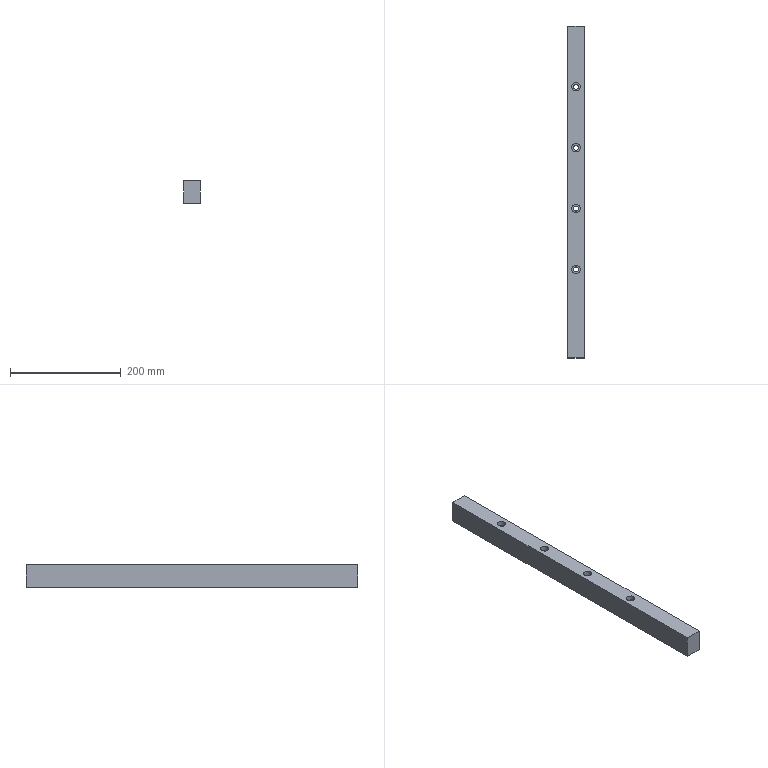Component | SolidWorks | GuideRailSpacer122-1 | 1 solid | 26 faces | box 30 x 600 x 41 mm | volume 723676 mm3 | cylinder 16 | plane 10 | commonest cylinder face diameters 15 x8 9 x8
build123d program:
from build123d import *

# Parameters (mm, degrees)
SKETCH1_W                                       = 30
SKETCH1_H                                       = 600
BOSS_EXTRUDE1_DEPTH                             = 41
M8_HEX_SOCKET_HEAD_CAP_SCREW_CBORE1_D           = 9
M8_HEX_SOCKET_HEAD_CAP_SCREW_CBORE1_CBORE_D     = 15
M8_HEX_SOCKET_HEAD_CAP_SCREW_CBORE1_CBORE_DEPTH = 8.6


with BuildPart() as part:
    # Sketch1 → Boss-Extrude1 (new body)
    with BuildSketch(Plane.XY):
        Rectangle(SKETCH1_W, SKETCH1_H)
    extrude(amount=BOSS_EXTRUDE1_DEPTH)

    # M8 Hex Socket Head Cap Screw CBORE1 (through all)
    with Locations(Plane.XY.offset(41)):
        with Locations((0, 190), (0, 80), (0, -30), (0, -140)):
            CounterBoreHole(M8_HEX_SOCKET_HEAD_CAP_SCREW_CBORE1_D / 2, M8_HEX_SOCKET_HEAD_CAP_SCREW_CBORE1_CBORE_D / 2, M8_HEX_SOCKET_HEAD_CAP_SCREW_CBORE1_CBORE_DEPTH)


solid = part.part

# Placed as in the assembly
solid = solid.moved(Location((-294.479, 164.741, 805), (0, 0, 0)))
STEP:
#1=COLOUR_RGB('',0.7922,0.8196,0.9333);
#2=FILL_AREA_STYLE_COLOUR('',#1);
#3=FILL_AREA_STYLE('',(#2));
#4=SURFACE_STYLE_FILL_AREA(#3);
#5=SURFACE_SIDE_STYLE('',(#4));
#6=SURFACE_STYLE_USAGE(.BOTH.,#5);
#7=PRESENTATION_STYLE_ASSIGNMENT((#6));
#8=CARTESIAN_POINT('',(-11.889,13.966,32.969));
#9=VERTEX_POINT('',#8);
#10=CARTESIAN_POINT('',(-11.298,13.966,32.969));
#11=VERTEX_POINT('',#10);
#12=CARTESIAN_POINT('',(-11.594,13.966,32.969));
#13=DIRECTION('',(0.,0.,1.));
#14=DIRECTION('',(1.,0.,0.));
#15=AXIS2_PLACEMENT_3D('',#12,#13,#14);
#16=CIRCLE('',#15,0.2953);
#17=EDGE_CURVE('',#9,#11,#16,.T.);
#18=ORIENTED_EDGE('',*,*,#17,.F.);
#19=CARTESIAN_POINT('',(-11.889,13.966,33.307));
#20=VERTEX_POINT('',#19);
#21=CARTESIAN_POINT('',(-11.889,13.966,33.307));
#22=DIRECTION('',(0.,0.,1.));
#23=VECTOR('',#22,39.37);
#24=LINE('',#21,#23);
#25=EDGE_CURVE('',#9,#20,#24,.T.);
#26=ORIENTED_EDGE('',*,*,#25,.T.);
#27=CARTESIAN_POINT('',(-11.298,13.966,33.307));
#28=VERTEX_POINT('',#27);
#29=CARTESIAN_POINT('',(-11.594,13.966,33.307));
#30=DIRECTION('',(0.,0.,1.));
#31=DIRECTION('',(1.,0.,0.));
#32=AXIS2_PLACEMENT_3D('',#29,#30,#31);
#33=CIRCLE('',#32,0.2953);
#34=EDGE_CURVE('',#20,#28,#33,.T.);
#35=ORIENTED_EDGE('',*,*,#34,.T.);
#36=CARTESIAN_POINT('',(-11.298,13.966,33.307));
#37=DIRECTION('',(0.,0.,1.));
#38=VECTOR('',#37,39.37);
#39=LINE('',#36,#38);
#40=EDGE_CURVE('',#11,#28,#39,.T.);
#41=ORIENTED_EDGE('',*,*,#40,.F.);
#42=EDGE_LOOP('',(#18,#26,#35,#41));
#43=FACE_OUTER_BOUND('',#42,.T.);
#44=CARTESIAN_POINT('',(-11.594,13.966,33.307));
#45=DIRECTION('',(0.,0.,1.));
#46=DIRECTION('',(1.,0.,0.));
#47=AXIS2_PLACEMENT_3D('',#44,#45,#46);
#48=CYLINDRICAL_SURFACE('',#47,0.2953);
#49=ADVANCED_FACE('',(#43),#48,.F.);
#50=CARTESIAN_POINT('',(-11.771,13.966,31.693));
#51=VERTEX_POINT('',#50);
#52=CARTESIAN_POINT('',(-11.416,13.966,31.693));
#53=VERTEX_POINT('',#52);
#54=CARTESIAN_POINT('',(-11.594,13.966,31.693));
#55=DIRECTION('',(0.,0.,1.));
#56=DIRECTION('',(1.,0.,0.));
#57=AXIS2_PLACEMENT_3D('',#54,#55,#56);
#58=CIRCLE('',#57,0.1772);
#59=EDGE_CURVE('',#51,#53,#58,.T.);
#60=ORIENTED_EDGE('',*,*,#59,.F.);
#61=CARTESIAN_POINT('',(-11.771,13.966,32.969));
#62=VERTEX_POINT('',#61);
#63=CARTESIAN_POINT('',(-11.771,13.966,33.307));
#64=DIRECTION('',(0.,0.,1.));
#65=VECTOR('',#64,39.37);
#66=LINE('',#63,#65);
#67=EDGE_CURVE('',#51,#62,#66,.T.);
#68=ORIENTED_EDGE('',*,*,#67,.T.);
#69=CARTESIAN_POINT('',(-11.416,13.966,32.969));
#70=VERTEX_POINT('',#69);
#71=CARTESIAN_POINT('',(-11.594,13.966,32.969));
#72=DIRECTION('',(0.,0.,1.));
#73=DIRECTION('',(1.,0.,0.));
#74=AXIS2_PLACEMENT_3D('',#71,#72,#73);
#75=CIRCLE('',#74,0.1772);
#76=EDGE_CURVE('',#62,#70,#75,.T.);
#77=ORIENTED_EDGE('',*,*,#76,.T.);
#78=CARTESIAN_POINT('',(-11.416,13.966,33.307));
#79=DIRECTION('',(0.,0.,1.));
#80=VECTOR('',#79,39.37);
#81=LINE('',#78,#80);
#82=EDGE_CURVE('',#53,#70,#81,.T.);
#83=ORIENTED_EDGE('',*,*,#82,.F.);
#84=EDGE_LOOP('',(#60,#68,#77,#83));
#85=FACE_OUTER_BOUND('',#84,.T.);
#86=CARTESIAN_POINT('',(-11.594,13.966,33.307));
#87=DIRECTION('',(0.,0.,1.));
#88=DIRECTION('',(1.,0.,0.));
#89=AXIS2_PLACEMENT_3D('',#86,#87,#88);
#90=CYLINDRICAL_SURFACE('',#89,0.1772);
#91=ADVANCED_FACE('',(#85),#90,.F.);
#92=CARTESIAN_POINT('',(-11.889,9.635,32.969));
#93=VERTEX_POINT('',#92);
#94=CARTESIAN_POINT('',(-11.298,9.635,32.969));
#95=VERTEX_POINT('',#94);
#96=CARTESIAN_POINT('',(-11.594,9.635,32.969));
#97=DIRECTION('',(0.,0.,1.));
#98=DIRECTION('',(1.,0.,0.));
#99=AXIS2_PLACEMENT_3D('',#96,#97,#98);
#100=CIRCLE('',#99,0.2953);
#101=EDGE_CURVE('',#93,#95,#100,.T.);
#102=ORIENTED_EDGE('',*,*,#101,.F.);
#103=CARTESIAN_POINT('',(-11.889,9.635,33.307));
#104=VERTEX_POINT('',#103);
#105=CARTESIAN_POINT('',(-11.889,9.635,33.307));
#106=DIRECTION('',(0.,0.,1.));
#107=VECTOR('',#106,39.37);
#108=LINE('',#105,#107);
#109=EDGE_CURVE('',#93,#104,#108,.T.);
#110=ORIENTED_EDGE('',*,*,#109,.T.);
#111=CARTESIAN_POINT('',(-11.298,9.635,33.307));
#112=VERTEX_POINT('',#111);
#113=CARTESIAN_POINT('',(-11.594,9.635,33.307));
#114=DIRECTION('',(0.,0.,1.));
#115=DIRECTION('',(1.,0.,0.));
#116=AXIS2_PLACEMENT_3D('',#113,#114,#115);
#117=CIRCLE('',#116,0.2953);
#118=EDGE_CURVE('',#104,#112,#117,.T.);
#119=ORIENTED_EDGE('',*,*,#118,.T.);
#120=CARTESIAN_POINT('',(-11.298,9.635,33.307));
#121=DIRECTION('',(0.,0.,1.));
#122=VECTOR('',#121,39.37);
#123=LINE('',#120,#122);
#124=EDGE_CURVE('',#95,#112,#123,.T.);
#125=ORIENTED_EDGE('',*,*,#124,.F.);
#126=EDGE_LOOP('',(#102,#110,#119,#125));
#127=FACE_OUTER_BOUND('',#126,.T.);
#128=CARTESIAN_POINT('',(-11.594,9.635,33.307));
#129=DIRECTION('',(0.,0.,1.));
#130=DIRECTION('',(1.,0.,0.));
#131=AXIS2_PLACEMENT_3D('',#128,#129,#130);
#132=CYLINDRICAL_SURFACE('',#131,0.2953);
#133=ADVANCED_FACE('',(#127),#132,.F.);
#134=CARTESIAN_POINT('',(-11.771,9.635,31.693));
#135=VERTEX_POINT('',#134);
#136=CARTESIAN_POINT('',(-11.416,9.635,31.693));
#137=VERTEX_POINT('',#136);
#138=CARTESIAN_POINT('',(-11.594,9.635,31.693));
#139=DIRECTION('',(0.,0.,1.));
#140=DIRECTION('',(1.,0.,0.));
#141=AXIS2_PLACEMENT_3D('',#138,#139,#140);
#142=CIRCLE('',#141,0.1772);
#143=EDGE_CURVE('',#135,#137,#142,.T.);
#144=ORIENTED_EDGE('',*,*,#143,.F.);
#145=CARTESIAN_POINT('',(-11.771,9.635,32.969));
#146=VERTEX_POINT('',#145);
#147=CARTESIAN_POINT('',(-11.771,9.635,33.307));
#148=DIRECTION('',(0.,0.,1.));
#149=VECTOR('',#148,39.37);
#150=LINE('',#147,#149);
#151=EDGE_CURVE('',#135,#146,#150,.T.);
#152=ORIENTED_EDGE('',*,*,#151,.T.);
#153=CARTESIAN_POINT('',(-11.416,9.635,32.969));
#154=VERTEX_POINT('',#153);
#155=CARTESIAN_POINT('',(-11.594,9.635,32.969));
#156=DIRECTION('',(0.,0.,1.));
#157=DIRECTION('',(1.,0.,0.));
#158=AXIS2_PLACEMENT_3D('',#155,#156,#157);
#159=CIRCLE('',#158,0.1772);
#160=EDGE_CURVE('',#146,#154,#159,.T.);
#161=ORIENTED_EDGE('',*,*,#160,.T.);
#162=CARTESIAN_POINT('',(-11.416,9.635,33.307));
#163=DIRECTION('',(0.,0.,1.));
#164=VECTOR('',#163,39.37);
#165=LINE('',#162,#164);
#166=EDGE_CURVE('',#137,#154,#165,.T.);
#167=ORIENTED_EDGE('',*,*,#166,.F.);
#168=EDGE_LOOP('',(#144,#152,#161,#167));
#169=FACE_OUTER_BOUND('',#168,.T.);
#170=CARTESIAN_POINT('',(-11.594,9.635,33.307));
#171=DIRECTION('',(0.,0.,1.));
#172=DIRECTION('',(1.,0.,0.));
#173=AXIS2_PLACEMENT_3D('',#170,#171,#172);
#174=CYLINDRICAL_SURFACE('',#173,0.1772);
#175=ADVANCED_FACE('',(#169),#174,.F.);
#176=CARTESIAN_POINT('',(-11.889,5.305,32.969));
#177=VERTEX_POINT('',#176);
#178=CARTESIAN_POINT('',(-11.298,5.305,32.969));
#179=VERTEX_POINT('',#178);
#180=CARTESIAN_POINT('',(-11.594,5.305,32.969));
#181=DIRECTION('',(0.,0.,1.));
#182=DIRECTION('',(1.,0.,0.));
#183=AXIS2_PLACEMENT_3D('',#180,#181,#182);
#184=CIRCLE('',#183,0.2953);
#185=EDGE_CURVE('',#177,#179,#184,.T.);
#186=ORIENTED_EDGE('',*,*,#185,.F.);
#187=CARTESIAN_POINT('',(-11.889,5.305,33.307));
#188=VERTEX_POINT('',#187);
#189=CARTESIAN_POINT('',(-11.889,5.305,33.307));
#190=DIRECTION('',(0.,0.,1.));
#191=VECTOR('',#190,39.37);
#192=LINE('',#189,#191);
#193=EDGE_CURVE('',#177,#188,#192,.T.);
#194=ORIENTED_EDGE('',*,*,#193,.T.);
#195=CARTESIAN_POINT('',(-11.298,5.305,33.307));
#196=VERTEX_POINT('',#195);
#197=CARTESIAN_POINT('',(-11.594,5.305,33.307));
#198=DIRECTION('',(0.,0.,1.));
#199=DIRECTION('',(1.,0.,0.));
#200=AXIS2_PLACEMENT_3D('',#197,#198,#199);
#201=CIRCLE('',#200,0.2953);
#202=EDGE_CURVE('',#188,#196,#201,.T.);
#203=ORIENTED_EDGE('',*,*,#202,.T.);
#204=CARTESIAN_POINT('',(-11.298,5.305,33.307));
#205=DIRECTION('',(0.,0.,1.));
#206=VECTOR('',#205,39.37);
#207=LINE('',#204,#206);
#208=EDGE_CURVE('',#179,#196,#207,.T.);
#209=ORIENTED_EDGE('',*,*,#208,.F.);
#210=EDGE_LOOP('',(#186,#194,#203,#209));
#211=FACE_OUTER_BOUND('',#210,.T.);
#212=CARTESIAN_POINT('',(-11.594,5.305,33.307));
#213=DIRECTION('',(0.,0.,1.));
#214=DIRECTION('',(1.,0.,0.));
#215=AXIS2_PLACEMENT_3D('',#212,#213,#214);
#216=CYLINDRICAL_SURFACE('',#215,0.2953);
#217=ADVANCED_FACE('',(#211),#216,.F.);
#218=CARTESIAN_POINT('',(-11.771,5.305,31.693));
#219=VERTEX_POINT('',#218);
#220=CARTESIAN_POINT('',(-11.416,5.305,31.693));
#221=VERTEX_POINT('',#220);
#222=CARTESIAN_POINT('',(-11.594,5.305,31.693));
#223=DIRECTION('',(0.,0.,1.));
#224=DIRECTION('',(1.,0.,0.));
#225=AXIS2_PLACEMENT_3D('',#222,#223,#224);
#226=CIRCLE('',#225,0.1772);
#227=EDGE_CURVE('',#219,#221,#226,.T.);
#228=ORIENTED_EDGE('',*,*,#227,.F.);
#229=CARTESIAN_POINT('',(-11.771,5.305,32.969));
#230=VERTEX_POINT('',#229);
#231=CARTESIAN_POINT('',(-11.771,5.305,33.307));
#232=DIRECTION('',(0.,0.,1.));
#233=VECTOR('',#232,39.37);
#234=LINE('',#231,#233);
#235=EDGE_CURVE('',#219,#230,#234,.T.);
#236=ORIENTED_EDGE('',*,*,#235,.T.);
#237=CARTESIAN_POINT('',(-11.416,5.305,32.969));
#238=VERTEX_POINT('',#237);
#239=CARTESIAN_POINT('',(-11.594,5.305,32.969));
#240=DIRECTION('',(0.,0.,1.));
#241=DIRECTION('',(1.,0.,0.));
#242=AXIS2_PLACEMENT_3D('',#239,#240,#241);
#243=CIRCLE('',#242,0.1772);
#244=EDGE_CURVE('',#230,#238,#243,.T.);
#245=ORIENTED_EDGE('',*,*,#244,.T.);
#246=CARTESIAN_POINT('',(-11.416,5.305,33.307));
#247=DIRECTION('',(0.,0.,1.));
#248=VECTOR('',#247,39.37);
#249=LINE('',#246,#248);
#250=EDGE_CURVE('',#221,#238,#249,.T.);
#251=ORIENTED_EDGE('',*,*,#250,.F.);
#252=EDGE_LOOP('',(#228,#236,#245,#251));
#253=FACE_OUTER_BOUND('',#252,.T.);
#254=CARTESIAN_POINT('',(-11.594,5.305,33.307));
#255=DIRECTION('',(0.,0.,1.));
#256=DIRECTION('',(1.,0.,0.));
#257=AXIS2_PLACEMENT_3D('',#254,#255,#256);
#258=CYLINDRICAL_SURFACE('',#257,0.1772);
#259=ADVANCED_FACE('',(#253),#258,.F.);
#260=CARTESIAN_POINT('',(-11.889,0.974,32.969));
#261=VERTEX_POINT('',#260);
#262=CARTESIAN_POINT('',(-11.298,0.974,32.969));
#263=VERTEX_POINT('',#262);
#264=CARTESIAN_POINT('',(-11.594,0.974,32.969));
#265=DIRECTION('',(0.,0.,1.));
#266=DIRECTION('',(1.,0.,0.));
#267=AXIS2_PLACEMENT_3D('',#264,#265,#266);
#268=CIRCLE('',#267,0.2953);
#269=EDGE_CURVE('',#261,#263,#268,.T.);
#270=ORIENTED_EDGE('',*,*,#269,.F.);
#271=CARTESIAN_POINT('',(-11.889,0.974,33.307));
#272=VERTEX_POINT('',#271);
#273=CARTESIAN_POINT('',(-11.889,0.974,33.307));
#274=DIRECTION('',(0.,0.,1.));
#275=VECTOR('',#274,39.37);
#276=LINE('',#273,#275);
#277=EDGE_CURVE('',#261,#272,#276,.T.);
#278=ORIENTED_EDGE('',*,*,#277,.T.);
#279=CARTESIAN_POINT('',(-11.298,0.974,33.307));
#280=VERTEX_POINT('',#279);
#281=CARTESIAN_POINT('',(-11.594,0.974,33.307));
#282=DIRECTION('',(0.,0.,1.));
#283=DIRECTION('',(1.,0.,0.));
#284=AXIS2_PLACEMENT_3D('',#281,#282,#283);
#285=CIRCLE('',#284,0.2953);
#286=EDGE_CURVE('',#272,#280,#285,.T.);
#287=ORIENTED_EDGE('',*,*,#286,.T.);
#288=CARTESIAN_POINT('',(-11.298,0.974,33.307));
#289=DIRECTION('',(0.,0.,1.));
#290=VECTOR('',#289,39.37);
#291=LINE('',#288,#290);
#292=EDGE_CURVE('',#263,#280,#291,.T.);
#293=ORIENTED_EDGE('',*,*,#292,.F.);
#294=EDGE_LOOP('',(#270,#278,#287,#293));
#295=FACE_OUTER_BOUND('',#294,.T.);
#296=CARTESIAN_POINT('',(-11.594,0.974,33.307));
#297=DIRECTION('',(0.,0.,1.));
#298=DIRECTION('',(1.,0.,0.));
#299=AXIS2_PLACEMENT_3D('',#296,#297,#298);
#300=CYLINDRICAL_SURFACE('',#299,0.2953);
#301=ADVANCED_FACE('',(#295),#300,.F.);
#302=CARTESIAN_POINT('',(-11.771,0.974,31.693));
#303=VERTEX_POINT('',#302);
#304=CARTESIAN_POINT('',(-11.416,0.974,31.693));
#305=VERTEX_POINT('',#304);
#306=CARTESIAN_POINT('',(-11.594,0.974,31.693));
#307=DIRECTION('',(0.,0.,1.));
#308=DIRECTION('',(1.,0.,0.));
#309=AXIS2_PLACEMENT_3D('',#306,#307,#308);
#310=CIRCLE('',#309,0.1772);
#311=EDGE_CURVE('',#303,#305,#310,.T.);
#312=ORIENTED_EDGE('',*,*,#311,.F.);
#313=CARTESIAN_POINT('',(-11.771,0.974,32.969));
#314=VERTEX_POINT('',#313);
#315=CARTESIAN_POINT('',(-11.771,0.974,33.307));
#316=DIRECTION('',(0.,0.,1.));
#317=VECTOR('',#316,39.37);
#318=LINE('',#315,#317);
#319=EDGE_CURVE('',#303,#314,#318,.T.);
#320=ORIENTED_EDGE('',*,*,#319,.T.);
#321=CARTESIAN_POINT('',(-11.416,0.974,32.969));
#322=VERTEX_POINT('',#321);
#323=CARTESIAN_POINT('',(-11.594,0.974,32.969));
#324=DIRECTION('',(0.,0.,1.));
#325=DIRECTION('',(1.,0.,0.));
#326=AXIS2_PLACEMENT_3D('',#323,#324,#325);
#327=CIRCLE('',#326,0.1772);
#328=EDGE_CURVE('',#314,#322,#327,.T.);
#329=ORIENTED_EDGE('',*,*,#328,.T.);
#330=CARTESIAN_POINT('',(-11.416,0.974,33.307));
#331=DIRECTION('',(0.,0.,1.));
#332=VECTOR('',#331,39.37);
#333=LINE('',#330,#332);
#334=EDGE_CURVE('',#305,#322,#333,.T.);
#335=ORIENTED_EDGE('',*,*,#334,.F.);
#336=EDGE_LOOP('',(#312,#320,#329,#335));
#337=FACE_OUTER_BOUND('',#336,.T.);
#338=CARTESIAN_POINT('',(-11.594,0.974,33.307));
#339=DIRECTION('',(0.,0.,1.));
#340=DIRECTION('',(1.,0.,0.));
#341=AXIS2_PLACEMENT_3D('',#338,#339,#340);
#342=CYLINDRICAL_SURFACE('',#341,0.1772);
#343=ADVANCED_FACE('',(#337),#342,.F.);
#344=CARTESIAN_POINT('',(-11.003,-5.325,31.693));
#345=VERTEX_POINT('',#344);
#346=CARTESIAN_POINT('',(-11.003,18.297,31.693));
#347=VERTEX_POINT('',#346);
#348=CARTESIAN_POINT('',(-11.003,-5.325,31.693));
#349=DIRECTION('',(0.,1.,0.));
#350=VECTOR('',#349,39.37);
#351=LINE('',#348,#350);
#352=EDGE_CURVE('',#345,#347,#351,.T.);
#353=ORIENTED_EDGE('',*,*,#352,.T.);
#354=CARTESIAN_POINT('',(-11.003,18.297,33.307));
#355=VERTEX_POINT('',#354);
#356=CARTESIAN_POINT('',(-11.003,18.297,33.307));
#357=DIRECTION('',(0.,0.,-1.));
#358=VECTOR('',#357,39.37);
#359=LINE('',#356,#358);
#360=EDGE_CURVE('',#355,#347,#359,.T.);
#361=ORIENTED_EDGE('',*,*,#360,.F.);
#362=CARTESIAN_POINT('',(-11.003,-5.325,33.307));
#363=VERTEX_POINT('',#362);
#364=CARTESIAN_POINT('',(-11.003,-5.325,33.307));
#365=DIRECTION('',(0.,1.,0.));
#366=VECTOR('',#365,39.37);
#367=LINE('',#364,#366);
#368=EDGE_CURVE('',#363,#355,#367,.T.);
#369=ORIENTED_EDGE('',*,*,#368,.F.);
#370=CARTESIAN_POINT('',(-11.003,-5.325,33.307));
#371=DIRECTION('',(0.,0.,-1.));
#372=VECTOR('',#371,39.37);
#373=LINE('',#370,#372);
#374=EDGE_CURVE('',#363,#345,#373,.T.);
#375=ORIENTED_EDGE('',*,*,#374,.T.);
#376=EDGE_LOOP('',(#353,#361,#369,#375));
#377=FACE_OUTER_BOUND('',#376,.T.);
#378=CARTESIAN_POINT('',(-11.003,-5.325,33.307));
#379=DIRECTION('',(-1.,0.,0.));
#380=DIRECTION('',(0.,0.,1.));
#381=AXIS2_PLACEMENT_3D('',#378,#379,#380);
#382=PLANE('',#381);
#383=ADVANCED_FACE('',(#377),#382,.F.);
#384=CARTESIAN_POINT('',(-12.184,18.297,31.693));
#385=VERTEX_POINT('',#384);
#386=CARTESIAN_POINT('',(-12.184,18.297,31.693));
#387=DIRECTION('',(-1.,0.,0.));
#388=VECTOR('',#387,39.37);
#389=LINE('',#386,#388);
#390=EDGE_CURVE('',#347,#385,#389,.T.);
#391=ORIENTED_EDGE('',*,*,#390,.T.);
#392=CARTESIAN_POINT('',(-12.184,18.297,33.307));
#393=VERTEX_POINT('',#392);
#394=CARTESIAN_POINT('',(-12.184,18.297,33.307));
#395=DIRECTION('',(0.,0.,-1.));
#396=VECTOR('',#395,39.37);
#397=LINE('',#394,#396);
#398=EDGE_CURVE('',#393,#385,#397,.T.);
#399=ORIENTED_EDGE('',*,*,#398,.F.);
#400=CARTESIAN_POINT('',(-12.184,18.297,33.307));
#401=DIRECTION('',(-1.,0.,0.));
#402=VECTOR('',#401,39.37);
#403=LINE('',#400,#402);
#404=EDGE_CURVE('',#355,#393,#403,.T.);
#405=ORIENTED_EDGE('',*,*,#404,.F.);
#406=ORIENTED_EDGE('',*,*,#360,.T.);
#407=EDGE_LOOP('',(#391,#399,#405,#406));
#408=FACE_OUTER_BOUND('',#407,.T.);
#409=CARTESIAN_POINT('',(-12.184,18.297,33.307));
#410=DIRECTION('',(0.,-1.,0.));
#411=DIRECTION('',(0.,0.,-1.));
#412=AXIS2_PLACEMENT_3D('',#409,#410,#411);
#413=PLANE('',#412);
#414=ADVANCED_FACE('',(#408),#413,.F.);
#415=CARTESIAN_POINT('',(-12.184,-5.325,31.693));
#416=VERTEX_POINT('',#415);
#417=CARTESIAN_POINT('',(-12.184,-5.325,31.693));
#418=DIRECTION('',(0.,-1.,0.));
#419=VECTOR('',#418,39.37);
#420=LINE('',#417,#419);
#421=EDGE_CURVE('',#385,#416,#420,.T.);
#422=ORIENTED_EDGE('',*,*,#421,.T.);
#423=CARTESIAN_POINT('',(-12.184,-5.325,33.307));
#424=VERTEX_POINT('',#423);
#425=CARTESIAN_POINT('',(-12.184,-5.325,33.307));
#426=DIRECTION('',(0.,0.,-1.));
#427=VECTOR('',#426,39.37);
#428=LINE('',#425,#427);
#429=EDGE_CURVE('',#424,#416,#428,.T.);
#430=ORIENTED_EDGE('',*,*,#429,.F.);
#431=CARTESIAN_POINT('',(-12.184,-5.325,33.307));
#432=DIRECTION('',(0.,-1.,0.));
#433=VECTOR('',#432,39.37);
#434=LINE('',#431,#433);
#435=EDGE_CURVE('',#393,#424,#434,.T.);
#436=ORIENTED_EDGE('',*,*,#435,.F.);
#437=ORIENTED_EDGE('',*,*,#398,.T.);
#438=EDGE_LOOP('',(#422,#430,#436,#437));
#439=FACE_OUTER_BOUND('',#438,.T.);
#440=CARTESIAN_POINT('',(-12.184,-5.325,33.307));
#441=DIRECTION('',(1.,0.,0.));
#442=DIRECTION('',(0.,0.,-1.));
#443=AXIS2_PLACEMENT_3D('',#440,#441,#442);
#444=PLANE('',#443);
#445=ADVANCED_FACE('',(#439),#444,.F.);
#446=CARTESIAN_POINT('',(-12.184,-5.325,31.693));
#447=DIRECTION('',(1.,0.,0.));
#448=VECTOR('',#447,39.37);
#449=LINE('',#446,#448);
#450=EDGE_CURVE('',#416,#345,#449,.T.);
#451=ORIENTED_EDGE('',*,*,#450,.T.);
#452=ORIENTED_EDGE('',*,*,#374,.F.);
#453=CARTESIAN_POINT('',(-12.184,-5.325,33.307));
#454=DIRECTION('',(1.,0.,0.));
#455=VECTOR('',#454,39.37);
#456=LINE('',#453,#455);
#457=EDGE_CURVE('',#424,#363,#456,.T.);
#458=ORIENTED_EDGE('',*,*,#457,.F.);
#459=ORIENTED_EDGE('',*,*,#429,.T.);
#460=EDGE_LOOP('',(#451,#452,#458,#459));
#461=FACE_OUTER_BOUND('',#460,.T.);
#462=CARTESIAN_POINT('',(-12.184,-5.325,33.307));
#463=DIRECTION('',(0.,1.,0.));
#464=DIRECTION('',(0.,0.,1.));
#465=AXIS2_PLACEMENT_3D('',#462,#463,#464);
#466=PLANE('',#465);
#467=ADVANCED_FACE('',(#461),#466,.F.);
#468=CARTESIAN_POINT('',(-11.594,13.966,33.307));
#469=DIRECTION('',(0.,0.,1.));
#470=DIRECTION('',(1.,0.,0.));
#471=AXIS2_PLACEMENT_3D('',#468,#469,#470);
#472=CIRCLE('',#471,0.2953);
#473=EDGE_CURVE('',#28,#20,#472,.T.);
#474=ORIENTED_EDGE('',*,*,#473,.F.);
#475=ORIENTED_EDGE('',*,*,#34,.F.);
#476=EDGE_LOOP('',(#474,#475));
#477=FACE_BOUND('',#476,.T.);
#478=CARTESIAN_POINT('',(-11.594,9.635,33.307));
#479=DIRECTION('',(0.,0.,1.));
#480=DIRECTION('',(1.,0.,0.));
#481=AXIS2_PLACEMENT_3D('',#478,#479,#480);
#482=CIRCLE('',#481,0.2953);
#483=EDGE_CURVE('',#112,#104,#482,.T.);
#484=ORIENTED_EDGE('',*,*,#483,.F.);
#485=ORIENTED_EDGE('',*,*,#118,.F.);
#486=EDGE_LOOP('',(#484,#485));
#487=FACE_BOUND('',#486,.T.);
#488=CARTESIAN_POINT('',(-11.594,5.305,33.307));
#489=DIRECTION('',(0.,0.,1.));
#490=DIRECTION('',(1.,0.,0.));
#491=AXIS2_PLACEMENT_3D('',#488,#489,#490);
#492=CIRCLE('',#491,0.2953);
#493=EDGE_CURVE('',#196,#188,#492,.T.);
#494=ORIENTED_EDGE('',*,*,#493,.F.);
#495=ORIENTED_EDGE('',*,*,#202,.F.);
#496=EDGE_LOOP('',(#494,#495));
#497=FACE_BOUND('',#496,.T.);
#498=CARTESIAN_POINT('',(-11.594,0.974,33.307));
#499=DIRECTION('',(0.,0.,1.));
#500=DIRECTION('',(1.,0.,0.));
#501=AXIS2_PLACEMENT_3D('',#498,#499,#500);
#502=CIRCLE('',#501,0.2953);
#503=EDGE_CURVE('',#280,#272,#502,.T.);
#504=ORIENTED_EDGE('',*,*,#503,.F.);
#505=ORIENTED_EDGE('',*,*,#286,.F.);
#506=EDGE_LOOP('',(#504,#505));
#507=FACE_BOUND('',#506,.T.);
#508=ORIENTED_EDGE('',*,*,#368,.T.);
#509=ORIENTED_EDGE('',*,*,#404,.T.);
#510=ORIENTED_EDGE('',*,*,#435,.T.);
#511=ORIENTED_EDGE('',*,*,#457,.T.);
#512=EDGE_LOOP('',(#508,#509,#510,#511));
#513=FACE_OUTER_BOUND('',#512,.T.);
#514=CARTESIAN_POINT('',(-11.594,6.486,33.307));
#515=DIRECTION('',(0.,0.,-1.));
#516=DIRECTION('',(-1.,0.,0.));
#517=AXIS2_PLACEMENT_3D('',#514,#515,#516);
#518=PLANE('',#517);
#519=ADVANCED_FACE('',(#477,#487,#497,#507,#513),#518,.F.);
#520=CARTESIAN_POINT('',(-11.594,13.966,31.693));
#521=DIRECTION('',(0.,0.,1.));
#522=DIRECTION('',(1.,0.,0.));
#523=AXIS2_PLACEMENT_3D('',#520,#521,#522);
#524=CIRCLE('',#523,0.1772);
#525=EDGE_CURVE('',#53,#51,#524,.T.);
#526=ORIENTED_EDGE('',*,*,#525,.T.);
#527=ORIENTED_EDGE('',*,*,#59,.T.);
#528=EDGE_LOOP('',(#526,#527));
#529=FACE_BOUND('',#528,.T.);
#530=CARTESIAN_POINT('',(-11.594,9.635,31.693));
#531=DIRECTION('',(0.,0.,1.));
#532=DIRECTION('',(1.,0.,0.));
#533=AXIS2_PLACEMENT_3D('',#530,#531,#532);
#534=CIRCLE('',#533,0.1772);
#535=EDGE_CURVE('',#137,#135,#534,.T.);
#536=ORIENTED_EDGE('',*,*,#535,.T.);
#537=ORIENTED_EDGE('',*,*,#143,.T.);
#538=EDGE_LOOP('',(#536,#537));
#539=FACE_BOUND('',#538,.T.);
#540=CARTESIAN_POINT('',(-11.594,5.305,31.693));
#541=DIRECTION('',(0.,0.,1.));
#542=DIRECTION('',(1.,0.,0.));
#543=AXIS2_PLACEMENT_3D('',#540,#541,#542);
#544=CIRCLE('',#543,0.1772);
#545=EDGE_CURVE('',#221,#219,#544,.T.);
#546=ORIENTED_EDGE('',*,*,#545,.T.);
#547=ORIENTED_EDGE('',*,*,#227,.T.);
#548=EDGE_LOOP('',(#546,#547));
#549=FACE_BOUND('',#548,.T.);
#550=CARTESIAN_POINT('',(-11.594,0.974,31.693));
#551=DIRECTION('',(0.,0.,1.));
#552=DIRECTION('',(1.,0.,0.));
#553=AXIS2_PLACEMENT_3D('',#550,#551,#552);
#554=CIRCLE('',#553,0.1772);
#555=EDGE_CURVE('',#305,#303,#554,.T.);
#556=ORIENTED_EDGE('',*,*,#555,.T.);
#557=ORIENTED_EDGE('',*,*,#311,.T.);
#558=EDGE_LOOP('',(#556,#557));
#559=FACE_BOUND('',#558,.T.);
#560=ORIENTED_EDGE('',*,*,#352,.F.);
#561=ORIENTED_EDGE('',*,*,#450,.F.);
#562=ORIENTED_EDGE('',*,*,#421,.F.);
#563=ORIENTED_EDGE('',*,*,#390,.F.);
#564=EDGE_LOOP('',(#560,#561,#562,#563));
#565=FACE_OUTER_BOUND('',#564,.T.);
#566=CARTESIAN_POINT('',(-11.594,6.486,31.693));
#567=DIRECTION('',(0.,0.,-1.));
#568=DIRECTION('',(-1.,0.,0.));
#569=AXIS2_PLACEMENT_3D('',#566,#567,#568);
#570=PLANE('',#569);
#571=ADVANCED_FACE('',(#529,#539,#549,#559,#565),#570,.T.);
#572=ORIENTED_EDGE('',*,*,#319,.F.);
#573=ORIENTED_EDGE('',*,*,#555,.F.);
#574=ORIENTED_EDGE('',*,*,#334,.T.);
#575=CARTESIAN_POINT('',(-11.594,0.974,32.969));
#576=DIRECTION('',(0.,0.,1.));
#577=DIRECTION('',(1.,0.,0.));
#578=AXIS2_PLACEMENT_3D('',#575,#576,#577);
#579=CIRCLE('',#578,0.1772);
#580=EDGE_CURVE('',#322,#314,#579,.T.);
#581=ORIENTED_EDGE('',*,*,#580,.T.);
#582=EDGE_LOOP('',(#572,#573,#574,#581));
#583=FACE_OUTER_BOUND('',#582,.T.);
#584=CARTESIAN_POINT('',(-11.594,0.974,33.307));
#585=DIRECTION('',(0.,0.,1.));
#586=DIRECTION('',(1.,0.,0.));
#587=AXIS2_PLACEMENT_3D('',#584,#585,#586);
#588=CYLINDRICAL_SURFACE('',#587,0.1772);
#589=ADVANCED_FACE('',(#583),#588,.F.);
#590=ORIENTED_EDGE('',*,*,#580,.F.);
#591=ORIENTED_EDGE('',*,*,#328,.F.);
#592=EDGE_LOOP('',(#590,#591));
#593=FACE_BOUND('',#592,.T.);
#594=CARTESIAN_POINT('',(-11.594,0.974,32.969));
#595=DIRECTION('',(0.,0.,1.));
#596=DIRECTION('',(1.,0.,0.));
#597=AXIS2_PLACEMENT_3D('',#594,#595,#596);
#598=CIRCLE('',#597,0.2953);
#599=EDGE_CURVE('',#263,#261,#598,.T.);
#600=ORIENTED_EDGE('',*,*,#599,.T.);
#601=ORIENTED_EDGE('',*,*,#269,.T.);
#602=EDGE_LOOP('',(#600,#601));
#603=FACE_OUTER_BOUND('',#602,.T.);
#604=CARTESIAN_POINT('',(-11.416,0.974,32.969));
#605=DIRECTION('',(0.,0.,-1.));
#606=DIRECTION('',(-1.,0.,0.));
#607=AXIS2_PLACEMENT_3D('',#604,#605,#606);
#608=PLANE('',#607);
#609=ADVANCED_FACE('',(#593,#603),#608,.F.);
#610=ORIENTED_EDGE('',*,*,#277,.F.);
#611=ORIENTED_EDGE('',*,*,#599,.F.);
#612=ORIENTED_EDGE('',*,*,#292,.T.);
#613=ORIENTED_EDGE('',*,*,#503,.T.);
#614=EDGE_LOOP('',(#610,#611,#612,#613));
#615=FACE_OUTER_BOUND('',#614,.T.);
#616=CARTESIAN_POINT('',(-11.594,0.974,33.307));
#617=DIRECTION('',(0.,0.,1.));
#618=DIRECTION('',(1.,0.,0.));
#619=AXIS2_PLACEMENT_3D('',#616,#617,#618);
#620=CYLINDRICAL_SURFACE('',#619,0.2953);
#621=ADVANCED_FACE('',(#615),#620,.F.);
#622=ORIENTED_EDGE('',*,*,#235,.F.);
#623=ORIENTED_EDGE('',*,*,#545,.F.);
#624=ORIENTED_EDGE('',*,*,#250,.T.);
#625=CARTESIAN_POINT('',(-11.594,5.305,32.969));
#626=DIRECTION('',(0.,0.,1.));
#627=DIRECTION('',(1.,0.,0.));
#628=AXIS2_PLACEMENT_3D('',#625,#626,#627);
#629=CIRCLE('',#628,0.1772);
#630=EDGE_CURVE('',#238,#230,#629,.T.);
#631=ORIENTED_EDGE('',*,*,#630,.T.);
#632=EDGE_LOOP('',(#622,#623,#624,#631));
#633=FACE_OUTER_BOUND('',#632,.T.);
#634=CARTESIAN_POINT('',(-11.594,5.305,33.307));
#635=DIRECTION('',(0.,0.,1.));
#636=DIRECTION('',(1.,0.,0.));
#637=AXIS2_PLACEMENT_3D('',#634,#635,#636);
#638=CYLINDRICAL_SURFACE('',#637,0.1772);
#639=ADVANCED_FACE('',(#633),#638,.F.);
#640=ORIENTED_EDGE('',*,*,#630,.F.);
#641=ORIENTED_EDGE('',*,*,#244,.F.);
#642=EDGE_LOOP('',(#640,#641));
#643=FACE_BOUND('',#642,.T.);
#644=CARTESIAN_POINT('',(-11.594,5.305,32.969));
#645=DIRECTION('',(0.,0.,1.));
#646=DIRECTION('',(1.,0.,0.));
#647=AXIS2_PLACEMENT_3D('',#644,#645,#646);
#648=CIRCLE('',#647,0.2953);
#649=EDGE_CURVE('',#179,#177,#648,.T.);
#650=ORIENTED_EDGE('',*,*,#649,.T.);
#651=ORIENTED_EDGE('',*,*,#185,.T.);
#652=EDGE_LOOP('',(#650,#651));
#653=FACE_OUTER_BOUND('',#652,.T.);
#654=CARTESIAN_POINT('',(-11.416,5.305,32.969));
#655=DIRECTION('',(0.,0.,-1.));
#656=DIRECTION('',(-1.,0.,0.));
#657=AXIS2_PLACEMENT_3D('',#654,#655,#656);
#658=PLANE('',#657);
#659=ADVANCED_FACE('',(#643,#653),#658,.F.);
#660=ORIENTED_EDGE('',*,*,#193,.F.);
#661=ORIENTED_EDGE('',*,*,#649,.F.);
#662=ORIENTED_EDGE('',*,*,#208,.T.);
#663=ORIENTED_EDGE('',*,*,#493,.T.);
#664=EDGE_LOOP('',(#660,#661,#662,#663));
#665=FACE_OUTER_BOUND('',#664,.T.);
#666=CARTESIAN_POINT('',(-11.594,5.305,33.307));
#667=DIRECTION('',(0.,0.,1.));
#668=DIRECTION('',(1.,0.,0.));
#669=AXIS2_PLACEMENT_3D('',#666,#667,#668);
#670=CYLINDRICAL_SURFACE('',#669,0.2953);
#671=ADVANCED_FACE('',(#665),#670,.F.);
#672=ORIENTED_EDGE('',*,*,#151,.F.);
#673=ORIENTED_EDGE('',*,*,#535,.F.);
#674=ORIENTED_EDGE('',*,*,#166,.T.);
#675=CARTESIAN_POINT('',(-11.594,9.635,32.969));
#676=DIRECTION('',(0.,0.,1.));
#677=DIRECTION('',(1.,0.,0.));
#678=AXIS2_PLACEMENT_3D('',#675,#676,#677);
#679=CIRCLE('',#678,0.1772);
#680=EDGE_CURVE('',#154,#146,#679,.T.);
#681=ORIENTED_EDGE('',*,*,#680,.T.);
#682=EDGE_LOOP('',(#672,#673,#674,#681));
#683=FACE_OUTER_BOUND('',#682,.T.);
#684=CARTESIAN_POINT('',(-11.594,9.635,33.307));
#685=DIRECTION('',(0.,0.,1.));
#686=DIRECTION('',(1.,0.,0.));
#687=AXIS2_PLACEMENT_3D('',#684,#685,#686);
#688=CYLINDRICAL_SURFACE('',#687,0.1772);
#689=ADVANCED_FACE('',(#683),#688,.F.);
#690=ORIENTED_EDGE('',*,*,#680,.F.);
#691=ORIENTED_EDGE('',*,*,#160,.F.);
#692=EDGE_LOOP('',(#690,#691));
#693=FACE_BOUND('',#692,.T.);
#694=CARTESIAN_POINT('',(-11.594,9.635,32.969));
#695=DIRECTION('',(0.,0.,1.));
#696=DIRECTION('',(1.,0.,0.));
#697=AXIS2_PLACEMENT_3D('',#694,#695,#696);
#698=CIRCLE('',#697,0.2953);
#699=EDGE_CURVE('',#95,#93,#698,.T.);
#700=ORIENTED_EDGE('',*,*,#699,.T.);
#701=ORIENTED_EDGE('',*,*,#101,.T.);
#702=EDGE_LOOP('',(#700,#701));
#703=FACE_OUTER_BOUND('',#702,.T.);
#704=CARTESIAN_POINT('',(-11.416,9.635,32.969));
#705=DIRECTION('',(0.,0.,-1.));
#706=DIRECTION('',(-1.,0.,0.));
#707=AXIS2_PLACEMENT_3D('',#704,#705,#706);
#708=PLANE('',#707);
#709=ADVANCED_FACE('',(#693,#703),#708,.F.);
#710=ORIENTED_EDGE('',*,*,#109,.F.);
#711=ORIENTED_EDGE('',*,*,#699,.F.);
#712=ORIENTED_EDGE('',*,*,#124,.T.);
#713=ORIENTED_EDGE('',*,*,#483,.T.);
#714=EDGE_LOOP('',(#710,#711,#712,#713));
#715=FACE_OUTER_BOUND('',#714,.T.);
#716=CARTESIAN_POINT('',(-11.594,9.635,33.307));
#717=DIRECTION('',(0.,0.,1.));
#718=DIRECTION('',(1.,0.,0.));
#719=AXIS2_PLACEMENT_3D('',#716,#717,#718);
#720=CYLINDRICAL_SURFACE('',#719,0.2953);
#721=ADVANCED_FACE('',(#715),#720,.F.);
#722=ORIENTED_EDGE('',*,*,#67,.F.);
#723=ORIENTED_EDGE('',*,*,#525,.F.);
#724=ORIENTED_EDGE('',*,*,#82,.T.);
#725=CARTESIAN_POINT('',(-11.594,13.966,32.969));
#726=DIRECTION('',(0.,0.,1.));
#727=DIRECTION('',(1.,0.,0.));
#728=AXIS2_PLACEMENT_3D('',#725,#726,#727);
#729=CIRCLE('',#728,0.1772);
#730=EDGE_CURVE('',#70,#62,#729,.T.);
#731=ORIENTED_EDGE('',*,*,#730,.T.);
#732=EDGE_LOOP('',(#722,#723,#724,#731));
#733=FACE_OUTER_BOUND('',#732,.T.);
#734=CARTESIAN_POINT('',(-11.594,13.966,33.307));
#735=DIRECTION('',(0.,0.,1.));
#736=DIRECTION('',(1.,0.,0.));
#737=AXIS2_PLACEMENT_3D('',#734,#735,#736);
#738=CYLINDRICAL_SURFACE('',#737,0.1772);
#739=ADVANCED_FACE('',(#733),#738,.F.);
#740=ORIENTED_EDGE('',*,*,#730,.F.);
#741=ORIENTED_EDGE('',*,*,#76,.F.);
#742=EDGE_LOOP('',(#740,#741));
#743=FACE_BOUND('',#742,.T.);
#744=CARTESIAN_POINT('',(-11.594,13.966,32.969));
#745=DIRECTION('',(0.,0.,1.));
#746=DIRECTION('',(1.,0.,0.));
#747=AXIS2_PLACEMENT_3D('',#744,#745,#746);
#748=CIRCLE('',#747,0.2953);
#749=EDGE_CURVE('',#11,#9,#748,.T.);
#750=ORIENTED_EDGE('',*,*,#749,.T.);
#751=ORIENTED_EDGE('',*,*,#17,.T.);
#752=EDGE_LOOP('',(#750,#751));
#753=FACE_OUTER_BOUND('',#752,.T.);
#754=CARTESIAN_POINT('',(-11.416,13.966,32.969));
#755=DIRECTION('',(0.,0.,-1.));
#756=DIRECTION('',(-1.,0.,0.));
#757=AXIS2_PLACEMENT_3D('',#754,#755,#756);
#758=PLANE('',#757);
#759=ADVANCED_FACE('',(#743,#753),#758,.F.);
#760=ORIENTED_EDGE('',*,*,#25,.F.);
#761=ORIENTED_EDGE('',*,*,#749,.F.);
#762=ORIENTED_EDGE('',*,*,#40,.T.);
#763=ORIENTED_EDGE('',*,*,#473,.T.);
#764=EDGE_LOOP('',(#760,#761,#762,#763));
#765=FACE_OUTER_BOUND('',#764,.T.);
#766=CARTESIAN_POINT('',(-11.594,13.966,33.307));
#767=DIRECTION('',(0.,0.,1.));
#768=DIRECTION('',(1.,0.,0.));
#769=AXIS2_PLACEMENT_3D('',#766,#767,#768);
#770=CYLINDRICAL_SURFACE('',#769,0.2953);
#771=ADVANCED_FACE('',(#765),#770,.F.);
#772=CLOSED_SHELL('',(#49,#91,#133,#175,#217,#259,#301,#343,#383,#414,#445,#467,#519,#571,#589,#609,#621,#639,#659,#671,#689,#709,#721,#739,#759,#771));
#773=MANIFOLD_SOLID_BREP('',#772);
#774=STYLED_ITEM('',(#7),#773);
#775=(LENGTH_UNIT()NAMED_UNIT(*)SI_UNIT($,.METRE.));
#776=LENGTH_MEASURE_WITH_UNIT(LENGTH_MEASURE(0.0254),#775);
#777=DIMENSIONAL_EXPONENTS(1.,0.,0.,0.,0.,0.,0.);
#778=(CONVERSION_BASED_UNIT('',#776)LENGTH_UNIT()NAMED_UNIT(#777));
#779=UNCERTAINTY_MEASURE_WITH_UNIT(LENGTH_MEASURE(0.00001),#778,'','');
#780=(NAMED_UNIT(*)PLANE_ANGLE_UNIT()SI_UNIT($,.RADIAN.));
#781=(NAMED_UNIT(*)SI_UNIT($,.STERADIAN.)SOLID_ANGLE_UNIT());
#782=(GEOMETRIC_REPRESENTATION_CONTEXT(3)GLOBAL_UNCERTAINTY_ASSIGNED_CONTEXT((#779))GLOBAL_UNIT_ASSIGNED_CONTEXT((#778,#780,#781))REPRESENTATION_CONTEXT('',''));
#783=MECHANICAL_DESIGN_GEOMETRIC_PRESENTATION_REPRESENTATION('',(#774),#782);
#784=CARTESIAN_POINT('',(0.,0.,0.));
#785=DIRECTION('',(0.,0.,1.));
#786=DIRECTION('',(1.,0.,0.));
#787=AXIS2_PLACEMENT_3D('',#784,#785,#786);
#788=(LENGTH_UNIT()NAMED_UNIT(*)SI_UNIT($,.METRE.));
#789=LENGTH_MEASURE_WITH_UNIT(LENGTH_MEASURE(0.0254),#788);
#790=DIMENSIONAL_EXPONENTS(1.,0.,0.,0.,0.,0.,0.);
#791=(CONVERSION_BASED_UNIT('',#789)LENGTH_UNIT()NAMED_UNIT(#790));
#792=UNCERTAINTY_MEASURE_WITH_UNIT(LENGTH_MEASURE(0.00001),#791,'','');
#793=(NAMED_UNIT(*)PLANE_ANGLE_UNIT()SI_UNIT($,.RADIAN.));
#794=(NAMED_UNIT(*)SI_UNIT($,.STERADIAN.)SOLID_ANGLE_UNIT());
#795=(GEOMETRIC_REPRESENTATION_CONTEXT(3)GLOBAL_UNCERTAINTY_ASSIGNED_CONTEXT((#792))GLOBAL_UNIT_ASSIGNED_CONTEXT((#791,#793,#794))REPRESENTATION_CONTEXT('',''));
#796=ADVANCED_BREP_SHAPE_REPRESENTATION('',(#773,#787),#795);
#797=PRESENTATION_LAYER_ASSIGNMENT('','',(#774));